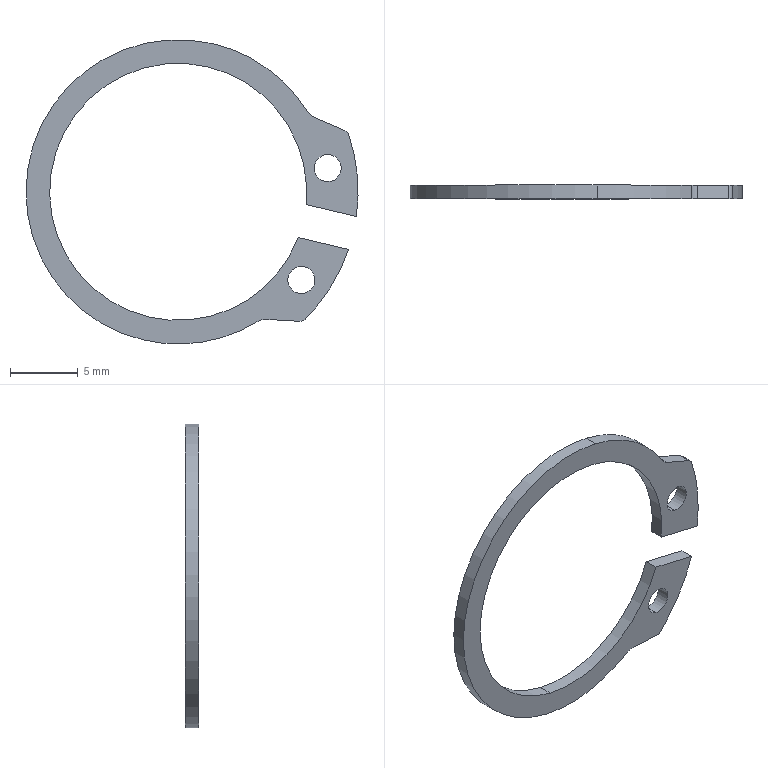Component | SolidWorks | ShaftRetainingRingTypeA-20-GB894.1-1986-2 | 1 solid | 22 faces | box 24.55 x 1 x 22.5 mm | volume 131 mm3 | cylinder 16 | plane 6 | commonest cylinder face diameters 2 x6 22.5 x3 19 x3 1 x2 26.6 x2 | material 65Mn
build123d program:
from build123d import *

# Parameters (mm, degrees)
BASE_EXTRUDE_DEPTH      = 0.5
BASE_EXTRUDE_DEPTH_BACK = 0.5
SKETCH1_R               = 1


with BuildPart() as part:
    # Sketch1 → Base-Extrude (new, two sides: drawn at the far end of the back side and taken through both)
    with BuildSketch(Plane.XY.offset(-BASE_EXTRUDE_DEPTH_BACK)):
        with BuildLine():
            Line((-1.25, -9.417), (-1.25, -13.241))
            ThreePointArc((-1.25, -13.241), (-4.249, -12.603), (-7.022, -11.295))
            ThreePointArc((-7.022, -11.295), (-7.172, -11.151), (-7.25, -10.958))
            Line((-7.25, -10.958), (-7.687, -8.479))
            ThreePointArc((-7.687, -8.479), (-7.785, -8.191), (-7.964, -7.946))
            ThreePointArc((-7.964, -7.946), (0, 11.25), (7.964, -7.946))
            ThreePointArc((7.964, -7.946), (7.785, -8.191), (7.687, -8.479))
            Line((7.687, -8.479), (7.25, -10.958))
            ThreePointArc((7.25, -10.958), (7.172, -11.151), (7.022, -11.295))
            ThreePointArc((7.022, -11.295), (4.249, -12.603), (1.25, -13.241))
            Line((1.25, -13.241), (1.25, -9.417))
            ThreePointArc((1.25, -9.417), (0, 9.5), (-1.25, -9.417))
        make_face()
        with Locations((-4.25, -10.362)):
            Circle(SKETCH1_R, mode=Mode.SUBTRACT)
        with Locations(Location((4.25, -10.362, 0), (0, 0, 180))):
            Circle(SKETCH1_R, mode=Mode.SUBTRACT)
    extrude(amount=BASE_EXTRUDE_DEPTH + BASE_EXTRUDE_DEPTH_BACK)


solid = part.part

# Placed as in the assembly
solid = solid.moved(Location((40.4, -163.15, 35), (-90, 0, 103.272)))
STEP:
#1=CARTESIAN_POINT('',(2.017,-6.443,1.409));
#2=VERTEX_POINT('',#1);
#3=CARTESIAN_POINT('',(2.035,-6.443,1.485));
#4=VERTEX_POINT('',#3);
#5=CARTESIAN_POINT('',(2.026,-6.443,1.447));
#6=DIRECTION('',(-0.,-1.,-0.));
#7=DIRECTION('',(-0.2296,0.,-0.9733));
#8=AXIS2_PLACEMENT_3D('',#5,#6,#7);
#9=CIRCLE('',#8,0.03937);
#10=EDGE_CURVE('',#2,#4,#9,.T.);
#11=ORIENTED_EDGE('',*,*,#10,.T.);
#12=CARTESIAN_POINT('',(2.035,-6.404,1.485));
#13=VERTEX_POINT('',#12);
#14=CARTESIAN_POINT('',(2.035,-6.443,1.485));
#15=DIRECTION('',(0.,1.,0.));
#16=VECTOR('',#15,39.37);
#17=LINE('',#14,#16);
#18=EDGE_CURVE('',#4,#13,#17,.T.);
#19=ORIENTED_EDGE('',*,*,#18,.T.);
#20=CARTESIAN_POINT('',(2.017,-6.404,1.409));
#21=VERTEX_POINT('',#20);
#22=CARTESIAN_POINT('',(2.026,-6.404,1.447));
#23=DIRECTION('',(-0.,-1.,-0.));
#24=DIRECTION('',(-0.2296,0.,-0.9733));
#25=AXIS2_PLACEMENT_3D('',#22,#23,#24);
#26=CIRCLE('',#25,0.03937);
#27=EDGE_CURVE('',#21,#13,#26,.T.);
#28=ORIENTED_EDGE('',*,*,#27,.F.);
#29=CARTESIAN_POINT('',(2.017,-6.443,1.409));
#30=DIRECTION('',(0.,1.,0.));
#31=VECTOR('',#30,39.37);
#32=LINE('',#29,#31);
#33=EDGE_CURVE('',#2,#21,#32,.T.);
#34=ORIENTED_EDGE('',*,*,#33,.F.);
#35=EDGE_LOOP('',(#11,#19,#28,#34));
#36=FACE_OUTER_BOUND('',#35,.T.);
#37=CARTESIAN_POINT('',(2.026,-6.443,1.447));
#38=DIRECTION('',(0.,1.,0.));
#39=DIRECTION('',(-0.2296,0.,-0.9733));
#40=AXIS2_PLACEMENT_3D('',#37,#38,#39);
#41=CYLINDRICAL_SURFACE('',#40,0.03937);
#42=ADVANCED_FACE('',(#36),#41,.F.);
#43=CARTESIAN_POINT('',(1.94,-6.443,1.083));
#44=VERTEX_POINT('',#43);
#45=CARTESIAN_POINT('',(1.958,-6.443,1.16));
#46=VERTEX_POINT('',#45);
#47=CARTESIAN_POINT('',(1.949,-6.443,1.121));
#48=DIRECTION('',(-0.,-1.,-0.));
#49=DIRECTION('',(0.2296,0.,0.9733));
#50=AXIS2_PLACEMENT_3D('',#47,#48,#49);
#51=CIRCLE('',#50,0.03937);
#52=EDGE_CURVE('',#44,#46,#51,.T.);
#53=ORIENTED_EDGE('',*,*,#52,.T.);
#54=CARTESIAN_POINT('',(1.958,-6.404,1.16));
#55=VERTEX_POINT('',#54);
#56=CARTESIAN_POINT('',(1.958,-6.443,1.16));
#57=DIRECTION('',(0.,1.,0.));
#58=VECTOR('',#57,39.37);
#59=LINE('',#56,#58);
#60=EDGE_CURVE('',#46,#55,#59,.T.);
#61=ORIENTED_EDGE('',*,*,#60,.T.);
#62=CARTESIAN_POINT('',(1.94,-6.404,1.083));
#63=VERTEX_POINT('',#62);
#64=CARTESIAN_POINT('',(1.949,-6.404,1.121));
#65=DIRECTION('',(-0.,-1.,-0.));
#66=DIRECTION('',(0.2296,0.,0.9733));
#67=AXIS2_PLACEMENT_3D('',#64,#65,#66);
#68=CIRCLE('',#67,0.03937);
#69=EDGE_CURVE('',#63,#55,#68,.T.);
#70=ORIENTED_EDGE('',*,*,#69,.F.);
#71=CARTESIAN_POINT('',(1.94,-6.443,1.083));
#72=DIRECTION('',(0.,1.,0.));
#73=VECTOR('',#72,39.37);
#74=LINE('',#71,#73);
#75=EDGE_CURVE('',#44,#63,#74,.T.);
#76=ORIENTED_EDGE('',*,*,#75,.F.);
#77=EDGE_LOOP('',(#53,#61,#70,#76));
#78=FACE_OUTER_BOUND('',#77,.T.);
#79=CARTESIAN_POINT('',(1.949,-6.443,1.121));
#80=DIRECTION('',(0.,1.,0.));
#81=DIRECTION('',(-0.2296,0.,-0.9733));
#82=AXIS2_PLACEMENT_3D('',#79,#80,#81);
#83=CYLINDRICAL_SURFACE('',#82,0.03937);
#84=ADVANCED_FACE('',(#78),#83,.F.);
#85=CARTESIAN_POINT('',(1.692,-6.443,1.809));
#86=VERTEX_POINT('',#85);
#87=CARTESIAN_POINT('',(1.489,-6.443,0.9469));
#88=VERTEX_POINT('',#87);
#89=CARTESIAN_POINT('',(1.591,-6.443,1.378));
#90=DIRECTION('',(-0.,-1.,-0.));
#91=DIRECTION('',(0.2296,0.,0.9733));
#92=AXIS2_PLACEMENT_3D('',#89,#90,#91);
#93=CIRCLE('',#92,0.4429);
#94=EDGE_CURVE('',#86,#88,#93,.T.);
#95=ORIENTED_EDGE('',*,*,#94,.F.);
#96=CARTESIAN_POINT('',(1.692,-6.404,1.809));
#97=VERTEX_POINT('',#96);
#98=CARTESIAN_POINT('',(1.692,-6.443,1.809));
#99=DIRECTION('',(0.,1.,0.));
#100=VECTOR('',#99,39.37);
#101=LINE('',#98,#100);
#102=EDGE_CURVE('',#86,#97,#101,.T.);
#103=ORIENTED_EDGE('',*,*,#102,.T.);
#104=CARTESIAN_POINT('',(1.489,-6.404,0.9469));
#105=VERTEX_POINT('',#104);
#106=CARTESIAN_POINT('',(1.591,-6.404,1.378));
#107=DIRECTION('',(-0.,-1.,-0.));
#108=DIRECTION('',(0.2296,0.,0.9733));
#109=AXIS2_PLACEMENT_3D('',#106,#107,#108);
#110=CIRCLE('',#109,0.4429);
#111=EDGE_CURVE('',#97,#105,#110,.T.);
#112=ORIENTED_EDGE('',*,*,#111,.T.);
#113=CARTESIAN_POINT('',(1.489,-6.443,0.9469));
#114=DIRECTION('',(0.,1.,0.));
#115=VECTOR('',#114,39.37);
#116=LINE('',#113,#115);
#117=EDGE_CURVE('',#88,#105,#116,.T.);
#118=ORIENTED_EDGE('',*,*,#117,.F.);
#119=EDGE_LOOP('',(#95,#103,#112,#118));
#120=FACE_OUTER_BOUND('',#119,.T.);
#121=CARTESIAN_POINT('',(1.591,-6.443,1.378));
#122=DIRECTION('',(0.,1.,0.));
#123=DIRECTION('',(-0.2296,0.,-0.9733));
#124=AXIS2_PLACEMENT_3D('',#121,#122,#123);
#125=CYLINDRICAL_SURFACE('',#124,0.4429);
#126=ADVANCED_FACE('',(#120),#125,.T.);
#127=CARTESIAN_POINT('',(1.823,-6.443,1.001));
#128=VERTEX_POINT('',#127);
#129=CARTESIAN_POINT('',(1.591,-6.443,1.378));
#130=DIRECTION('',(-0.,-1.,-0.));
#131=DIRECTION('',(0.2296,0.,0.9733));
#132=AXIS2_PLACEMENT_3D('',#129,#130,#131);
#133=CIRCLE('',#132,0.4429);
#134=EDGE_CURVE('',#88,#128,#133,.T.);
#135=ORIENTED_EDGE('',*,*,#134,.F.);
#136=ORIENTED_EDGE('',*,*,#117,.T.);
#137=CARTESIAN_POINT('',(1.823,-6.404,1.001));
#138=VERTEX_POINT('',#137);
#139=CARTESIAN_POINT('',(1.591,-6.404,1.378));
#140=DIRECTION('',(-0.,-1.,-0.));
#141=DIRECTION('',(0.2296,0.,0.9733));
#142=AXIS2_PLACEMENT_3D('',#139,#140,#141);
#143=CIRCLE('',#142,0.4429);
#144=EDGE_CURVE('',#105,#138,#143,.T.);
#145=ORIENTED_EDGE('',*,*,#144,.T.);
#146=CARTESIAN_POINT('',(1.823,-6.443,1.001));
#147=DIRECTION('',(0.,1.,0.));
#148=VECTOR('',#147,39.37);
#149=LINE('',#146,#148);
#150=EDGE_CURVE('',#128,#138,#149,.T.);
#151=ORIENTED_EDGE('',*,*,#150,.F.);
#152=EDGE_LOOP('',(#135,#136,#145,#151));
#153=FACE_OUTER_BOUND('',#152,.T.);
#154=CARTESIAN_POINT('',(1.591,-6.443,1.378));
#155=DIRECTION('',(0.,1.,0.));
#156=DIRECTION('',(-0.2296,0.,-0.9733));
#157=AXIS2_PLACEMENT_3D('',#154,#155,#156);
#158=CYLINDRICAL_SURFACE('',#157,0.4429);
#159=ADVANCED_FACE('',(#153),#158,.T.);
#160=CARTESIAN_POINT('',(1.676,-6.443,1.742));
#161=VERTEX_POINT('',#160);
#162=CARTESIAN_POINT('',(1.963,-6.443,1.341));
#163=VERTEX_POINT('',#162);
#164=CARTESIAN_POINT('',(1.591,-6.443,1.378));
#165=DIRECTION('',(0.,1.,0.));
#166=DIRECTION('',(0.2296,0.,0.9733));
#167=AXIS2_PLACEMENT_3D('',#164,#165,#166);
#168=CIRCLE('',#167,0.374);
#169=EDGE_CURVE('',#161,#163,#168,.T.);
#170=ORIENTED_EDGE('',*,*,#169,.F.);
#171=CARTESIAN_POINT('',(1.676,-6.404,1.742));
#172=VERTEX_POINT('',#171);
#173=CARTESIAN_POINT('',(1.676,-6.443,1.742));
#174=DIRECTION('',(0.,1.,0.));
#175=VECTOR('',#174,39.37);
#176=LINE('',#173,#175);
#177=EDGE_CURVE('',#161,#172,#176,.T.);
#178=ORIENTED_EDGE('',*,*,#177,.T.);
#179=CARTESIAN_POINT('',(1.963,-6.404,1.341));
#180=VERTEX_POINT('',#179);
#181=CARTESIAN_POINT('',(1.591,-6.404,1.378));
#182=DIRECTION('',(0.,1.,0.));
#183=DIRECTION('',(0.2296,0.,0.9733));
#184=AXIS2_PLACEMENT_3D('',#181,#182,#183);
#185=CIRCLE('',#184,0.374);
#186=EDGE_CURVE('',#172,#180,#185,.T.);
#187=ORIENTED_EDGE('',*,*,#186,.T.);
#188=CARTESIAN_POINT('',(1.963,-6.443,1.341));
#189=DIRECTION('',(0.,1.,0.));
#190=VECTOR('',#189,39.37);
#191=LINE('',#188,#190);
#192=EDGE_CURVE('',#163,#180,#191,.T.);
#193=ORIENTED_EDGE('',*,*,#192,.F.);
#194=EDGE_LOOP('',(#170,#178,#187,#193));
#195=FACE_OUTER_BOUND('',#194,.T.);
#196=CARTESIAN_POINT('',(1.591,-6.443,1.378));
#197=DIRECTION('',(0.,1.,0.));
#198=DIRECTION('',(-0.2296,0.,-0.9733));
#199=AXIS2_PLACEMENT_3D('',#196,#197,#198);
#200=CYLINDRICAL_SURFACE('',#199,0.374);
#201=ADVANCED_FACE('',(#195),#200,.F.);
#202=ORIENTED_EDGE('',*,*,#177,.F.);
#203=CARTESIAN_POINT('',(1.505,-6.443,1.014));
#204=VERTEX_POINT('',#203);
#205=CARTESIAN_POINT('',(1.591,-6.443,1.378));
#206=DIRECTION('',(0.,1.,0.));
#207=DIRECTION('',(0.2296,0.,0.9733));
#208=AXIS2_PLACEMENT_3D('',#205,#206,#207);
#209=CIRCLE('',#208,0.374);
#210=EDGE_CURVE('',#204,#161,#209,.T.);
#211=ORIENTED_EDGE('',*,*,#210,.F.);
#212=CARTESIAN_POINT('',(1.505,-6.404,1.014));
#213=VERTEX_POINT('',#212);
#214=CARTESIAN_POINT('',(1.505,-6.443,1.014));
#215=DIRECTION('',(0.,1.,0.));
#216=VECTOR('',#215,39.37);
#217=LINE('',#214,#216);
#218=EDGE_CURVE('',#204,#213,#217,.T.);
#219=ORIENTED_EDGE('',*,*,#218,.T.);
#220=CARTESIAN_POINT('',(1.591,-6.404,1.378));
#221=DIRECTION('',(0.,1.,0.));
#222=DIRECTION('',(0.2296,0.,0.9733));
#223=AXIS2_PLACEMENT_3D('',#220,#221,#222);
#224=CIRCLE('',#223,0.374);
#225=EDGE_CURVE('',#213,#172,#224,.T.);
#226=ORIENTED_EDGE('',*,*,#225,.T.);
#227=EDGE_LOOP('',(#202,#211,#219,#226));
#228=FACE_OUTER_BOUND('',#227,.T.);
#229=CARTESIAN_POINT('',(1.591,-6.443,1.378));
#230=DIRECTION('',(0.,1.,0.));
#231=DIRECTION('',(-0.2296,0.,-0.9733));
#232=AXIS2_PLACEMENT_3D('',#229,#230,#231);
#233=CYLINDRICAL_SURFACE('',#232,0.374);
#234=ADVANCED_FACE('',(#228),#233,.F.);
#235=ORIENTED_EDGE('',*,*,#52,.F.);
#236=CARTESIAN_POINT('',(1.949,-6.443,1.121));
#237=DIRECTION('',(-0.,-1.,-0.));
#238=DIRECTION('',(0.2296,0.,0.9733));
#239=AXIS2_PLACEMENT_3D('',#236,#237,#238);
#240=CIRCLE('',#239,0.03937);
#241=EDGE_CURVE('',#46,#44,#240,.T.);
#242=ORIENTED_EDGE('',*,*,#241,.F.);
#243=EDGE_LOOP('',(#235,#242));
#244=FACE_BOUND('',#243,.T.);
#245=CARTESIAN_POINT('',(1.846,-6.443,1.007));
#246=VERTEX_POINT('',#245);
#247=CARTESIAN_POINT('',(1.844,-6.443,0.9675));
#248=DIRECTION('',(0.,1.,0.));
#249=DIRECTION('',(0.2296,0.,0.9733));
#250=AXIS2_PLACEMENT_3D('',#247,#248,#249);
#251=CIRCLE('',#250,0.03937);
#252=EDGE_CURVE('',#128,#246,#251,.T.);
#253=ORIENTED_EDGE('',*,*,#252,.T.);
#254=CARTESIAN_POINT('',(1.945,-6.443,1.001));
#255=VERTEX_POINT('',#254);
#256=CARTESIAN_POINT('',(1.846,-6.443,1.007));
#257=DIRECTION('',(0.9984,-0.,-0.05708));
#258=VECTOR('',#257,39.37);
#259=LINE('',#256,#258);
#260=EDGE_CURVE('',#246,#255,#259,.T.);
#261=ORIENTED_EDGE('',*,*,#260,.T.);
#262=CARTESIAN_POINT('',(1.96,-6.443,1.007));
#263=VERTEX_POINT('',#262);
#264=CARTESIAN_POINT('',(1.946,-6.443,1.021));
#265=DIRECTION('',(-0.,-1.,-0.));
#266=DIRECTION('',(-0.2296,0.,-0.9733));
#267=AXIS2_PLACEMENT_3D('',#264,#265,#266);
#268=CIRCLE('',#267,0.01969);
#269=EDGE_CURVE('',#255,#263,#268,.T.);
#270=ORIENTED_EDGE('',*,*,#269,.T.);
#271=CARTESIAN_POINT('',(2.087,-6.443,1.21));
#272=VERTEX_POINT('',#271);
#273=CARTESIAN_POINT('',(1.591,-6.443,1.378));
#274=DIRECTION('',(-0.,-1.,-0.));
#275=DIRECTION('',(-0.2296,0.,-0.9733));
#276=AXIS2_PLACEMENT_3D('',#273,#274,#275);
#277=CIRCLE('',#276,0.5236);
#278=EDGE_CURVE('',#263,#272,#277,.T.);
#279=ORIENTED_EDGE('',*,*,#278,.T.);
#280=CARTESIAN_POINT('',(1.94,-6.443,1.245));
#281=VERTEX_POINT('',#280);
#282=CARTESIAN_POINT('',(1.94,-6.443,1.245));
#283=DIRECTION('',(-0.9733,0.,0.2296));
#284=VECTOR('',#283,39.37);
#285=LINE('',#282,#284);
#286=EDGE_CURVE('',#272,#281,#285,.T.);
#287=ORIENTED_EDGE('',*,*,#286,.T.);
#288=CARTESIAN_POINT('',(1.591,-6.443,1.378));
#289=DIRECTION('',(0.,1.,0.));
#290=DIRECTION('',(0.2296,0.,0.9733));
#291=AXIS2_PLACEMENT_3D('',#288,#289,#290);
#292=CIRCLE('',#291,0.374);
#293=EDGE_CURVE('',#281,#204,#292,.T.);
#294=ORIENTED_EDGE('',*,*,#293,.T.);
#295=ORIENTED_EDGE('',*,*,#210,.T.);
#296=ORIENTED_EDGE('',*,*,#169,.T.);
#297=CARTESIAN_POINT('',(2.109,-6.443,1.306));
#298=VERTEX_POINT('',#297);
#299=CARTESIAN_POINT('',(1.963,-6.443,1.341));
#300=DIRECTION('',(0.9733,-0.,-0.2296));
#301=VECTOR('',#300,39.37);
#302=LINE('',#299,#301);
#303=EDGE_CURVE('',#163,#298,#302,.T.);
#304=ORIENTED_EDGE('',*,*,#303,.T.);
#305=CARTESIAN_POINT('',(2.087,-6.443,1.545));
#306=VERTEX_POINT('',#305);
#307=CARTESIAN_POINT('',(1.591,-6.443,1.378));
#308=DIRECTION('',(-0.,-1.,-0.));
#309=DIRECTION('',(0.2296,0.,0.9733));
#310=AXIS2_PLACEMENT_3D('',#307,#308,#309);
#311=CIRCLE('',#310,0.5236);
#312=EDGE_CURVE('',#298,#306,#311,.T.);
#313=ORIENTED_EDGE('',*,*,#312,.T.);
#314=CARTESIAN_POINT('',(2.076,-6.443,1.557));
#315=VERTEX_POINT('',#314);
#316=CARTESIAN_POINT('',(2.068,-6.443,1.539));
#317=DIRECTION('',(-0.,-1.,-0.));
#318=DIRECTION('',(0.2296,0.,0.9733));
#319=AXIS2_PLACEMENT_3D('',#316,#317,#318);
#320=CIRCLE('',#319,0.01969);
#321=EDGE_CURVE('',#306,#315,#320,.T.);
#322=ORIENTED_EDGE('',*,*,#321,.T.);
#323=CARTESIAN_POINT('',(1.985,-6.443,1.596));
#324=VERTEX_POINT('',#323);
#325=CARTESIAN_POINT('',(1.985,-6.443,1.596));
#326=DIRECTION('',(-0.9186,0.,0.3951));
#327=VECTOR('',#326,39.37);
#328=LINE('',#325,#327);
#329=EDGE_CURVE('',#315,#324,#328,.T.);
#330=ORIENTED_EDGE('',*,*,#329,.T.);
#331=CARTESIAN_POINT('',(1.967,-6.443,1.611));
#332=VERTEX_POINT('',#331);
#333=CARTESIAN_POINT('',(2.,-6.443,1.632));
#334=DIRECTION('',(0.,1.,0.));
#335=DIRECTION('',(-0.2296,0.,-0.9733));
#336=AXIS2_PLACEMENT_3D('',#333,#334,#335);
#337=CIRCLE('',#336,0.03937);
#338=EDGE_CURVE('',#324,#332,#337,.T.);
#339=ORIENTED_EDGE('',*,*,#338,.T.);
#340=CARTESIAN_POINT('',(1.591,-6.443,1.378));
#341=DIRECTION('',(-0.,-1.,-0.));
#342=DIRECTION('',(0.2296,0.,0.9733));
#343=AXIS2_PLACEMENT_3D('',#340,#341,#342);
#344=CIRCLE('',#343,0.4429);
#345=EDGE_CURVE('',#332,#86,#344,.T.);
#346=ORIENTED_EDGE('',*,*,#345,.T.);
#347=ORIENTED_EDGE('',*,*,#94,.T.);
#348=ORIENTED_EDGE('',*,*,#134,.T.);
#349=EDGE_LOOP('',(#253,#261,#270,#279,#287,#294,#295,#296,#304,#313,#322,#330,#339,#346,#347,#348));
#350=FACE_OUTER_BOUND('',#349,.T.);
#351=ORIENTED_EDGE('',*,*,#10,.F.);
#352=CARTESIAN_POINT('',(2.026,-6.443,1.447));
#353=DIRECTION('',(-0.,-1.,-0.));
#354=DIRECTION('',(-0.2296,0.,-0.9733));
#355=AXIS2_PLACEMENT_3D('',#352,#353,#354);
#356=CIRCLE('',#355,0.03937);
#357=EDGE_CURVE('',#4,#2,#356,.T.);
#358=ORIENTED_EDGE('',*,*,#357,.F.);
#359=EDGE_LOOP('',(#351,#358));
#360=FACE_BOUND('',#359,.T.);
#361=CARTESIAN_POINT('',(1.844,-6.443,0.9675));
#362=DIRECTION('',(-0.,-1.,-0.));
#363=DIRECTION('',(0.2296,-0.,0.9733));
#364=AXIS2_PLACEMENT_3D('',#361,#362,#363);
#365=PLANE('',#364);
#366=ADVANCED_FACE('',(#244,#350,#360),#365,.T.);
#367=ORIENTED_EDGE('',*,*,#150,.T.);
#368=CARTESIAN_POINT('',(1.846,-6.404,1.007));
#369=VERTEX_POINT('',#368);
#370=CARTESIAN_POINT('',(1.844,-6.404,0.9675));
#371=DIRECTION('',(0.,1.,0.));
#372=DIRECTION('',(0.2296,0.,0.9733));
#373=AXIS2_PLACEMENT_3D('',#370,#371,#372);
#374=CIRCLE('',#373,0.03937);
#375=EDGE_CURVE('',#138,#369,#374,.T.);
#376=ORIENTED_EDGE('',*,*,#375,.T.);
#377=CARTESIAN_POINT('',(1.846,-6.443,1.007));
#378=DIRECTION('',(0.,1.,0.));
#379=VECTOR('',#378,39.37);
#380=LINE('',#377,#379);
#381=EDGE_CURVE('',#246,#369,#380,.T.);
#382=ORIENTED_EDGE('',*,*,#381,.F.);
#383=ORIENTED_EDGE('',*,*,#252,.F.);
#384=EDGE_LOOP('',(#367,#376,#382,#383));
#385=FACE_OUTER_BOUND('',#384,.T.);
#386=CARTESIAN_POINT('',(1.844,-6.443,0.9675));
#387=DIRECTION('',(0.,1.,0.));
#388=DIRECTION('',(-0.2296,0.,-0.9733));
#389=AXIS2_PLACEMENT_3D('',#386,#387,#388);
#390=CYLINDRICAL_SURFACE('',#389,0.03937);
#391=ADVANCED_FACE('',(#385),#390,.F.);
#392=ORIENTED_EDGE('',*,*,#381,.T.);
#393=CARTESIAN_POINT('',(1.945,-6.404,1.001));
#394=VERTEX_POINT('',#393);
#395=CARTESIAN_POINT('',(1.846,-6.404,1.007));
#396=DIRECTION('',(0.9984,-0.,-0.05708));
#397=VECTOR('',#396,39.37);
#398=LINE('',#395,#397);
#399=EDGE_CURVE('',#369,#394,#398,.T.);
#400=ORIENTED_EDGE('',*,*,#399,.T.);
#401=CARTESIAN_POINT('',(1.945,-6.443,1.001));
#402=DIRECTION('',(0.,1.,0.));
#403=VECTOR('',#402,39.37);
#404=LINE('',#401,#403);
#405=EDGE_CURVE('',#255,#394,#404,.T.);
#406=ORIENTED_EDGE('',*,*,#405,.F.);
#407=ORIENTED_EDGE('',*,*,#260,.F.);
#408=EDGE_LOOP('',(#392,#400,#406,#407));
#409=FACE_OUTER_BOUND('',#408,.T.);
#410=CARTESIAN_POINT('',(1.846,-6.443,1.007));
#411=DIRECTION('',(0.05708,-0.,0.9984));
#412=DIRECTION('',(-0.9984,0.,0.05708));
#413=AXIS2_PLACEMENT_3D('',#410,#411,#412);
#414=PLANE('',#413);
#415=ADVANCED_FACE('',(#409),#414,.F.);
#416=ORIENTED_EDGE('',*,*,#405,.T.);
#417=CARTESIAN_POINT('',(1.96,-6.404,1.007));
#418=VERTEX_POINT('',#417);
#419=CARTESIAN_POINT('',(1.946,-6.404,1.021));
#420=DIRECTION('',(-0.,-1.,-0.));
#421=DIRECTION('',(-0.2296,0.,-0.9733));
#422=AXIS2_PLACEMENT_3D('',#419,#420,#421);
#423=CIRCLE('',#422,0.01969);
#424=EDGE_CURVE('',#394,#418,#423,.T.);
#425=ORIENTED_EDGE('',*,*,#424,.T.);
#426=CARTESIAN_POINT('',(1.96,-6.443,1.007));
#427=DIRECTION('',(0.,1.,0.));
#428=VECTOR('',#427,39.37);
#429=LINE('',#426,#428);
#430=EDGE_CURVE('',#263,#418,#429,.T.);
#431=ORIENTED_EDGE('',*,*,#430,.F.);
#432=ORIENTED_EDGE('',*,*,#269,.F.);
#433=EDGE_LOOP('',(#416,#425,#431,#432));
#434=FACE_OUTER_BOUND('',#433,.T.);
#435=CARTESIAN_POINT('',(1.946,-6.443,1.021));
#436=DIRECTION('',(0.,1.,0.));
#437=DIRECTION('',(-0.2296,0.,-0.9733));
#438=AXIS2_PLACEMENT_3D('',#435,#436,#437);
#439=CYLINDRICAL_SURFACE('',#438,0.01969);
#440=ADVANCED_FACE('',(#434),#439,.T.);
#441=ORIENTED_EDGE('',*,*,#430,.T.);
#442=CARTESIAN_POINT('',(2.087,-6.404,1.21));
#443=VERTEX_POINT('',#442);
#444=CARTESIAN_POINT('',(1.591,-6.404,1.378));
#445=DIRECTION('',(-0.,-1.,-0.));
#446=DIRECTION('',(-0.2296,0.,-0.9733));
#447=AXIS2_PLACEMENT_3D('',#444,#445,#446);
#448=CIRCLE('',#447,0.5236);
#449=EDGE_CURVE('',#418,#443,#448,.T.);
#450=ORIENTED_EDGE('',*,*,#449,.T.);
#451=CARTESIAN_POINT('',(2.087,-6.443,1.21));
#452=DIRECTION('',(0.,1.,0.));
#453=VECTOR('',#452,39.37);
#454=LINE('',#451,#453);
#455=EDGE_CURVE('',#272,#443,#454,.T.);
#456=ORIENTED_EDGE('',*,*,#455,.F.);
#457=ORIENTED_EDGE('',*,*,#278,.F.);
#458=EDGE_LOOP('',(#441,#450,#456,#457));
#459=FACE_OUTER_BOUND('',#458,.T.);
#460=CARTESIAN_POINT('',(1.591,-6.443,1.378));
#461=DIRECTION('',(0.,1.,0.));
#462=DIRECTION('',(-0.2296,0.,-0.9733));
#463=AXIS2_PLACEMENT_3D('',#460,#461,#462);
#464=CYLINDRICAL_SURFACE('',#463,0.5236);
#465=ADVANCED_FACE('',(#459),#464,.T.);
#466=ORIENTED_EDGE('',*,*,#455,.T.);
#467=CARTESIAN_POINT('',(1.94,-6.404,1.245));
#468=VERTEX_POINT('',#467);
#469=CARTESIAN_POINT('',(1.94,-6.404,1.245));
#470=DIRECTION('',(-0.9733,0.,0.2296));
#471=VECTOR('',#470,39.37);
#472=LINE('',#469,#471);
#473=EDGE_CURVE('',#443,#468,#472,.T.);
#474=ORIENTED_EDGE('',*,*,#473,.T.);
#475=CARTESIAN_POINT('',(1.94,-6.443,1.245));
#476=DIRECTION('',(0.,1.,0.));
#477=VECTOR('',#476,39.37);
#478=LINE('',#475,#477);
#479=EDGE_CURVE('',#281,#468,#478,.T.);
#480=ORIENTED_EDGE('',*,*,#479,.F.);
#481=ORIENTED_EDGE('',*,*,#286,.F.);
#482=EDGE_LOOP('',(#466,#474,#480,#481));
#483=FACE_OUTER_BOUND('',#482,.T.);
#484=CARTESIAN_POINT('',(1.94,-6.443,1.245));
#485=DIRECTION('',(-0.2296,0.,-0.9733));
#486=DIRECTION('',(-0.,-1.,-0.));
#487=AXIS2_PLACEMENT_3D('',#484,#485,#486);
#488=PLANE('',#487);
#489=ADVANCED_FACE('',(#483),#488,.F.);
#490=ORIENTED_EDGE('',*,*,#218,.F.);
#491=ORIENTED_EDGE('',*,*,#293,.F.);
#492=ORIENTED_EDGE('',*,*,#479,.T.);
#493=CARTESIAN_POINT('',(1.591,-6.404,1.378));
#494=DIRECTION('',(0.,1.,0.));
#495=DIRECTION('',(0.2296,0.,0.9733));
#496=AXIS2_PLACEMENT_3D('',#493,#494,#495);
#497=CIRCLE('',#496,0.374);
#498=EDGE_CURVE('',#468,#213,#497,.T.);
#499=ORIENTED_EDGE('',*,*,#498,.T.);
#500=EDGE_LOOP('',(#490,#491,#492,#499));
#501=FACE_OUTER_BOUND('',#500,.T.);
#502=CARTESIAN_POINT('',(1.591,-6.443,1.378));
#503=DIRECTION('',(0.,1.,0.));
#504=DIRECTION('',(-0.2296,0.,-0.9733));
#505=AXIS2_PLACEMENT_3D('',#502,#503,#504);
#506=CYLINDRICAL_SURFACE('',#505,0.374);
#507=ADVANCED_FACE('',(#501),#506,.F.);
#508=ORIENTED_EDGE('',*,*,#192,.T.);
#509=CARTESIAN_POINT('',(2.109,-6.404,1.306));
#510=VERTEX_POINT('',#509);
#511=CARTESIAN_POINT('',(1.963,-6.404,1.341));
#512=DIRECTION('',(0.9733,-0.,-0.2296));
#513=VECTOR('',#512,39.37);
#514=LINE('',#511,#513);
#515=EDGE_CURVE('',#180,#510,#514,.T.);
#516=ORIENTED_EDGE('',*,*,#515,.T.);
#517=CARTESIAN_POINT('',(2.109,-6.443,1.306));
#518=DIRECTION('',(0.,1.,0.));
#519=VECTOR('',#518,39.37);
#520=LINE('',#517,#519);
#521=EDGE_CURVE('',#298,#510,#520,.T.);
#522=ORIENTED_EDGE('',*,*,#521,.F.);
#523=ORIENTED_EDGE('',*,*,#303,.F.);
#524=EDGE_LOOP('',(#508,#516,#522,#523));
#525=FACE_OUTER_BOUND('',#524,.T.);
#526=CARTESIAN_POINT('',(1.963,-6.443,1.341));
#527=DIRECTION('',(0.2296,-0.,0.9733));
#528=DIRECTION('',(-0.9733,0.,0.2296));
#529=AXIS2_PLACEMENT_3D('',#526,#527,#528);
#530=PLANE('',#529);
#531=ADVANCED_FACE('',(#525),#530,.F.);
#532=ORIENTED_EDGE('',*,*,#521,.T.);
#533=CARTESIAN_POINT('',(2.087,-6.404,1.545));
#534=VERTEX_POINT('',#533);
#535=CARTESIAN_POINT('',(1.591,-6.404,1.378));
#536=DIRECTION('',(-0.,-1.,-0.));
#537=DIRECTION('',(0.2296,0.,0.9733));
#538=AXIS2_PLACEMENT_3D('',#535,#536,#537);
#539=CIRCLE('',#538,0.5236);
#540=EDGE_CURVE('',#510,#534,#539,.T.);
#541=ORIENTED_EDGE('',*,*,#540,.T.);
#542=CARTESIAN_POINT('',(2.087,-6.443,1.545));
#543=DIRECTION('',(0.,1.,0.));
#544=VECTOR('',#543,39.37);
#545=LINE('',#542,#544);
#546=EDGE_CURVE('',#306,#534,#545,.T.);
#547=ORIENTED_EDGE('',*,*,#546,.F.);
#548=ORIENTED_EDGE('',*,*,#312,.F.);
#549=EDGE_LOOP('',(#532,#541,#547,#548));
#550=FACE_OUTER_BOUND('',#549,.T.);
#551=CARTESIAN_POINT('',(1.591,-6.443,1.378));
#552=DIRECTION('',(0.,1.,0.));
#553=DIRECTION('',(-0.2296,0.,-0.9733));
#554=AXIS2_PLACEMENT_3D('',#551,#552,#553);
#555=CYLINDRICAL_SURFACE('',#554,0.5236);
#556=ADVANCED_FACE('',(#550),#555,.T.);
#557=ORIENTED_EDGE('',*,*,#546,.T.);
#558=CARTESIAN_POINT('',(2.076,-6.404,1.557));
#559=VERTEX_POINT('',#558);
#560=CARTESIAN_POINT('',(2.068,-6.404,1.539));
#561=DIRECTION('',(-0.,-1.,-0.));
#562=DIRECTION('',(0.2296,0.,0.9733));
#563=AXIS2_PLACEMENT_3D('',#560,#561,#562);
#564=CIRCLE('',#563,0.01969);
#565=EDGE_CURVE('',#534,#559,#564,.T.);
#566=ORIENTED_EDGE('',*,*,#565,.T.);
#567=CARTESIAN_POINT('',(2.076,-6.443,1.557));
#568=DIRECTION('',(0.,1.,0.));
#569=VECTOR('',#568,39.37);
#570=LINE('',#567,#569);
#571=EDGE_CURVE('',#315,#559,#570,.T.);
#572=ORIENTED_EDGE('',*,*,#571,.F.);
#573=ORIENTED_EDGE('',*,*,#321,.F.);
#574=EDGE_LOOP('',(#557,#566,#572,#573));
#575=FACE_OUTER_BOUND('',#574,.T.);
#576=CARTESIAN_POINT('',(2.068,-6.443,1.539));
#577=DIRECTION('',(0.,1.,0.));
#578=DIRECTION('',(-0.2296,0.,-0.9733));
#579=AXIS2_PLACEMENT_3D('',#576,#577,#578);
#580=CYLINDRICAL_SURFACE('',#579,0.01969);
#581=ADVANCED_FACE('',(#575),#580,.T.);
#582=ORIENTED_EDGE('',*,*,#571,.T.);
#583=CARTESIAN_POINT('',(1.985,-6.404,1.596));
#584=VERTEX_POINT('',#583);
#585=CARTESIAN_POINT('',(1.985,-6.404,1.596));
#586=DIRECTION('',(-0.9186,0.,0.3951));
#587=VECTOR('',#586,39.37);
#588=LINE('',#585,#587);
#589=EDGE_CURVE('',#559,#584,#588,.T.);
#590=ORIENTED_EDGE('',*,*,#589,.T.);
#591=CARTESIAN_POINT('',(1.985,-6.443,1.596));
#592=DIRECTION('',(0.,1.,0.));
#593=VECTOR('',#592,39.37);
#594=LINE('',#591,#593);
#595=EDGE_CURVE('',#324,#584,#594,.T.);
#596=ORIENTED_EDGE('',*,*,#595,.F.);
#597=ORIENTED_EDGE('',*,*,#329,.F.);
#598=EDGE_LOOP('',(#582,#590,#596,#597));
#599=FACE_OUTER_BOUND('',#598,.T.);
#600=CARTESIAN_POINT('',(1.985,-6.443,1.596));
#601=DIRECTION('',(-0.3951,0.,-0.9186));
#602=DIRECTION('',(0.9186,-0.,-0.3951));
#603=AXIS2_PLACEMENT_3D('',#600,#601,#602);
#604=PLANE('',#603);
#605=ADVANCED_FACE('',(#599),#604,.F.);
#606=ORIENTED_EDGE('',*,*,#595,.T.);
#607=CARTESIAN_POINT('',(1.967,-6.404,1.611));
#608=VERTEX_POINT('',#607);
#609=CARTESIAN_POINT('',(2.,-6.404,1.632));
#610=DIRECTION('',(0.,1.,0.));
#611=DIRECTION('',(-0.2296,0.,-0.9733));
#612=AXIS2_PLACEMENT_3D('',#609,#610,#611);
#613=CIRCLE('',#612,0.03937);
#614=EDGE_CURVE('',#584,#608,#613,.T.);
#615=ORIENTED_EDGE('',*,*,#614,.T.);
#616=CARTESIAN_POINT('',(1.967,-6.443,1.611));
#617=DIRECTION('',(0.,1.,0.));
#618=VECTOR('',#617,39.37);
#619=LINE('',#616,#618);
#620=EDGE_CURVE('',#332,#608,#619,.T.);
#621=ORIENTED_EDGE('',*,*,#620,.F.);
#622=ORIENTED_EDGE('',*,*,#338,.F.);
#623=EDGE_LOOP('',(#606,#615,#621,#622));
#624=FACE_OUTER_BOUND('',#623,.T.);
#625=CARTESIAN_POINT('',(2.,-6.443,1.632));
#626=DIRECTION('',(0.,1.,0.));
#627=DIRECTION('',(-0.2296,0.,-0.9733));
#628=AXIS2_PLACEMENT_3D('',#625,#626,#627);
#629=CYLINDRICAL_SURFACE('',#628,0.03937);
#630=ADVANCED_FACE('',(#624),#629,.F.);
#631=ORIENTED_EDGE('',*,*,#102,.F.);
#632=ORIENTED_EDGE('',*,*,#345,.F.);
#633=ORIENTED_EDGE('',*,*,#620,.T.);
#634=CARTESIAN_POINT('',(1.591,-6.404,1.378));
#635=DIRECTION('',(-0.,-1.,-0.));
#636=DIRECTION('',(0.2296,0.,0.9733));
#637=AXIS2_PLACEMENT_3D('',#634,#635,#636);
#638=CIRCLE('',#637,0.4429);
#639=EDGE_CURVE('',#608,#97,#638,.T.);
#640=ORIENTED_EDGE('',*,*,#639,.T.);
#641=EDGE_LOOP('',(#631,#632,#633,#640));
#642=FACE_OUTER_BOUND('',#641,.T.);
#643=CARTESIAN_POINT('',(1.591,-6.443,1.378));
#644=DIRECTION('',(0.,1.,0.));
#645=DIRECTION('',(-0.2296,0.,-0.9733));
#646=AXIS2_PLACEMENT_3D('',#643,#644,#645);
#647=CYLINDRICAL_SURFACE('',#646,0.4429);
#648=ADVANCED_FACE('',(#642),#647,.T.);
#649=ORIENTED_EDGE('',*,*,#60,.F.);
#650=ORIENTED_EDGE('',*,*,#241,.T.);
#651=ORIENTED_EDGE('',*,*,#75,.T.);
#652=CARTESIAN_POINT('',(1.949,-6.404,1.121));
#653=DIRECTION('',(-0.,-1.,-0.));
#654=DIRECTION('',(0.2296,0.,0.9733));
#655=AXIS2_PLACEMENT_3D('',#652,#653,#654);
#656=CIRCLE('',#655,0.03937);
#657=EDGE_CURVE('',#55,#63,#656,.T.);
#658=ORIENTED_EDGE('',*,*,#657,.F.);
#659=EDGE_LOOP('',(#649,#650,#651,#658));
#660=FACE_OUTER_BOUND('',#659,.T.);
#661=CARTESIAN_POINT('',(1.949,-6.443,1.121));
#662=DIRECTION('',(0.,1.,0.));
#663=DIRECTION('',(-0.2296,0.,-0.9733));
#664=AXIS2_PLACEMENT_3D('',#661,#662,#663);
#665=CYLINDRICAL_SURFACE('',#664,0.03937);
#666=ADVANCED_FACE('',(#660),#665,.F.);
#667=ORIENTED_EDGE('',*,*,#18,.F.);
#668=ORIENTED_EDGE('',*,*,#357,.T.);
#669=ORIENTED_EDGE('',*,*,#33,.T.);
#670=CARTESIAN_POINT('',(2.026,-6.404,1.447));
#671=DIRECTION('',(-0.,-1.,-0.));
#672=DIRECTION('',(-0.2296,0.,-0.9733));
#673=AXIS2_PLACEMENT_3D('',#670,#671,#672);
#674=CIRCLE('',#673,0.03937);
#675=EDGE_CURVE('',#13,#21,#674,.T.);
#676=ORIENTED_EDGE('',*,*,#675,.F.);
#677=EDGE_LOOP('',(#667,#668,#669,#676));
#678=FACE_OUTER_BOUND('',#677,.T.);
#679=CARTESIAN_POINT('',(2.026,-6.443,1.447));
#680=DIRECTION('',(0.,1.,0.));
#681=DIRECTION('',(-0.2296,0.,-0.9733));
#682=AXIS2_PLACEMENT_3D('',#679,#680,#681);
#683=CYLINDRICAL_SURFACE('',#682,0.03937);
#684=ADVANCED_FACE('',(#678),#683,.F.);
#685=ORIENTED_EDGE('',*,*,#27,.T.);
#686=ORIENTED_EDGE('',*,*,#675,.T.);
#687=EDGE_LOOP('',(#685,#686));
#688=FACE_BOUND('',#687,.T.);
#689=ORIENTED_EDGE('',*,*,#69,.T.);
#690=ORIENTED_EDGE('',*,*,#657,.T.);
#691=EDGE_LOOP('',(#689,#690));
#692=FACE_BOUND('',#691,.T.);
#693=ORIENTED_EDGE('',*,*,#375,.F.);
#694=ORIENTED_EDGE('',*,*,#144,.F.);
#695=ORIENTED_EDGE('',*,*,#111,.F.);
#696=ORIENTED_EDGE('',*,*,#639,.F.);
#697=ORIENTED_EDGE('',*,*,#614,.F.);
#698=ORIENTED_EDGE('',*,*,#589,.F.);
#699=ORIENTED_EDGE('',*,*,#565,.F.);
#700=ORIENTED_EDGE('',*,*,#540,.F.);
#701=ORIENTED_EDGE('',*,*,#515,.F.);
#702=ORIENTED_EDGE('',*,*,#186,.F.);
#703=ORIENTED_EDGE('',*,*,#225,.F.);
#704=ORIENTED_EDGE('',*,*,#498,.F.);
#705=ORIENTED_EDGE('',*,*,#473,.F.);
#706=ORIENTED_EDGE('',*,*,#449,.F.);
#707=ORIENTED_EDGE('',*,*,#424,.F.);
#708=ORIENTED_EDGE('',*,*,#399,.F.);
#709=EDGE_LOOP('',(#693,#694,#695,#696,#697,#698,#699,#700,#701,#702,#703,#704,#705,#706,#707,#708));
#710=FACE_OUTER_BOUND('',#709,.T.);
#711=CARTESIAN_POINT('',(1.844,-6.404,0.9675));
#712=DIRECTION('',(-0.,-1.,-0.));
#713=DIRECTION('',(0.2296,-0.,0.9733));
#714=AXIS2_PLACEMENT_3D('',#711,#712,#713);
#715=PLANE('',#714);
#716=ADVANCED_FACE('',(#688,#692,#710),#715,.F.);
#717=CLOSED_SHELL('',(#42,#84,#126,#159,#201,#234,#366,#391,#415,#440,#465,#489,#507,#531,#556,#581,#605,#630,#648,#666,#684,#716));
#718=MANIFOLD_SOLID_BREP('',#717);
#719=CARTESIAN_POINT('',(0.,0.,0.));
#720=DIRECTION('',(0.,0.,1.));
#721=DIRECTION('',(1.,0.,0.));
#722=AXIS2_PLACEMENT_3D('',#719,#720,#721);
#723=(LENGTH_UNIT()NAMED_UNIT(*)SI_UNIT($,.METRE.));
#724=LENGTH_MEASURE_WITH_UNIT(LENGTH_MEASURE(0.0254),#723);
#725=DIMENSIONAL_EXPONENTS(1.,0.,0.,0.,0.,0.,0.);
#726=(CONVERSION_BASED_UNIT('',#724)LENGTH_UNIT()NAMED_UNIT(#725));
#727=UNCERTAINTY_MEASURE_WITH_UNIT(LENGTH_MEASURE(0.00001),#726,'','');
#728=(NAMED_UNIT(*)PLANE_ANGLE_UNIT()SI_UNIT($,.RADIAN.));
#729=(NAMED_UNIT(*)SI_UNIT($,.STERADIAN.)SOLID_ANGLE_UNIT());
#730=(GEOMETRIC_REPRESENTATION_CONTEXT(3)GLOBAL_UNCERTAINTY_ASSIGNED_CONTEXT((#727))GLOBAL_UNIT_ASSIGNED_CONTEXT((#726,#728,#729))REPRESENTATION_CONTEXT('',''));
#731=ADVANCED_BREP_SHAPE_REPRESENTATION('',(#718,#722),#730);
#732=COLOUR_RGB('',0.7922,0.8196,0.9333);
#733=FILL_AREA_STYLE_COLOUR('',#732);
#734=FILL_AREA_STYLE('',(#733));
#735=SURFACE_STYLE_FILL_AREA(#734);
#736=SURFACE_SIDE_STYLE('',(#735));
#737=SURFACE_STYLE_USAGE(.BOTH.,#736);
#738=PRESENTATION_STYLE_ASSIGNMENT((#737));
#739=STYLED_ITEM('',(#738),#718);
#740=(LENGTH_UNIT()NAMED_UNIT(*)SI_UNIT($,.METRE.));
#741=LENGTH_MEASURE_WITH_UNIT(LENGTH_MEASURE(0.0254),#740);
#742=DIMENSIONAL_EXPONENTS(1.,0.,0.,0.,0.,0.,0.);
#743=(CONVERSION_BASED_UNIT('',#741)LENGTH_UNIT()NAMED_UNIT(#742));
#744=UNCERTAINTY_MEASURE_WITH_UNIT(LENGTH_MEASURE(0.00001),#743,'','');
#745=(NAMED_UNIT(*)PLANE_ANGLE_UNIT()SI_UNIT($,.RADIAN.));
#746=(NAMED_UNIT(*)SI_UNIT($,.STERADIAN.)SOLID_ANGLE_UNIT());
#747=(GEOMETRIC_REPRESENTATION_CONTEXT(3)GLOBAL_UNCERTAINTY_ASSIGNED_CONTEXT((#744))GLOBAL_UNIT_ASSIGNED_CONTEXT((#743,#745,#746))REPRESENTATION_CONTEXT('',''));
#748=MECHANICAL_DESIGN_GEOMETRIC_PRESENTATION_REPRESENTATION('',(#739),#747);
#749=PRESENTATION_LAYER_ASSIGNMENT('','',(#739));